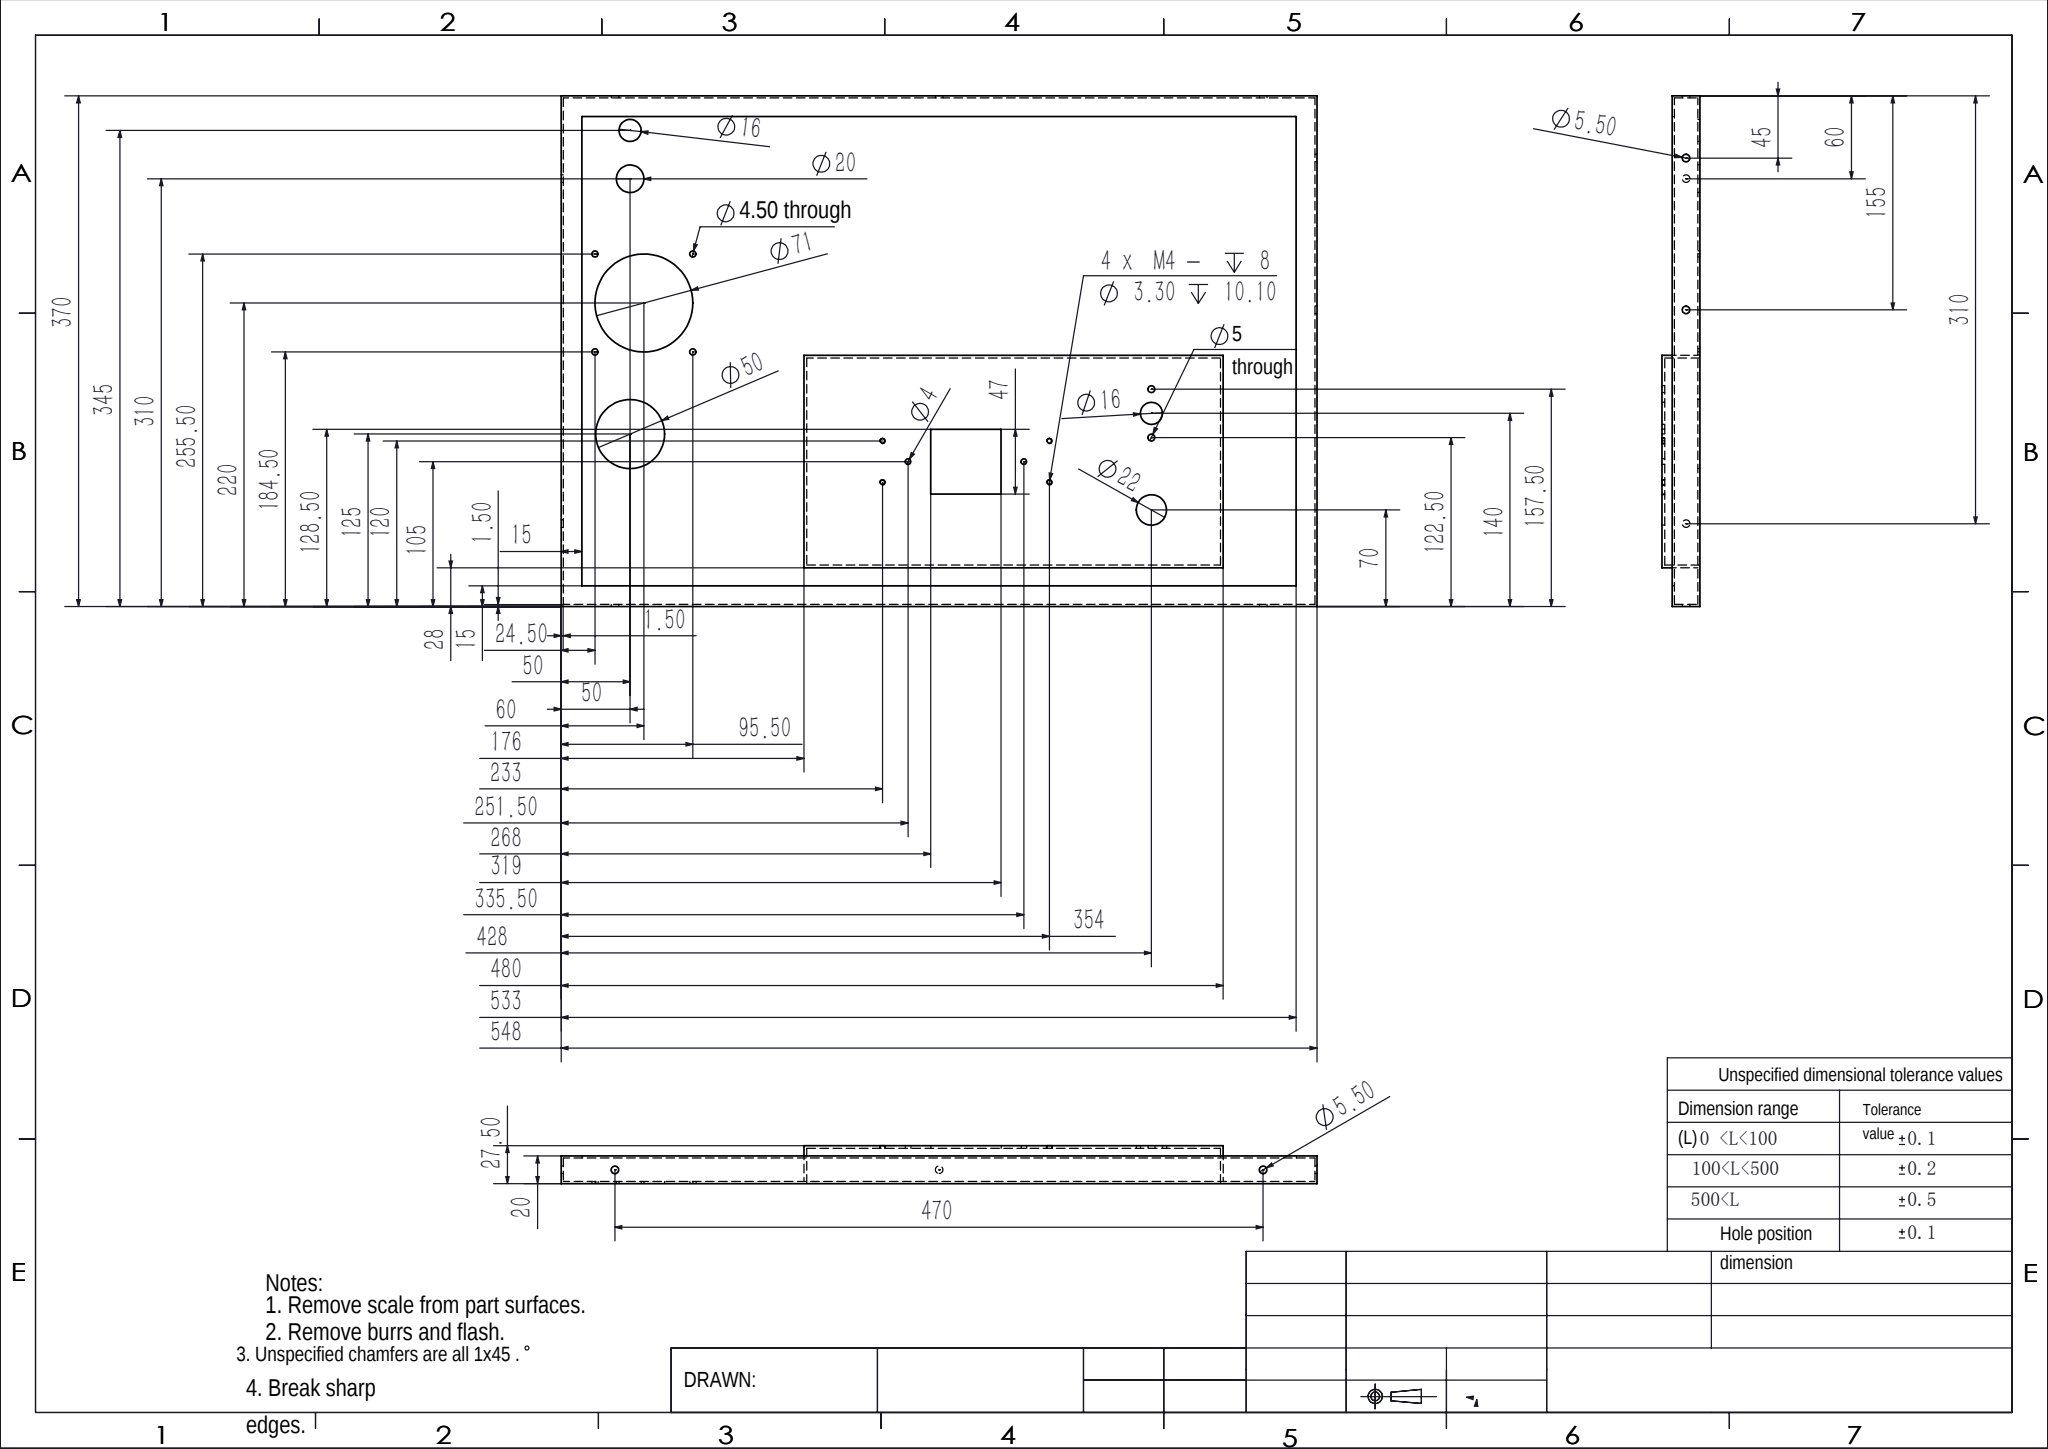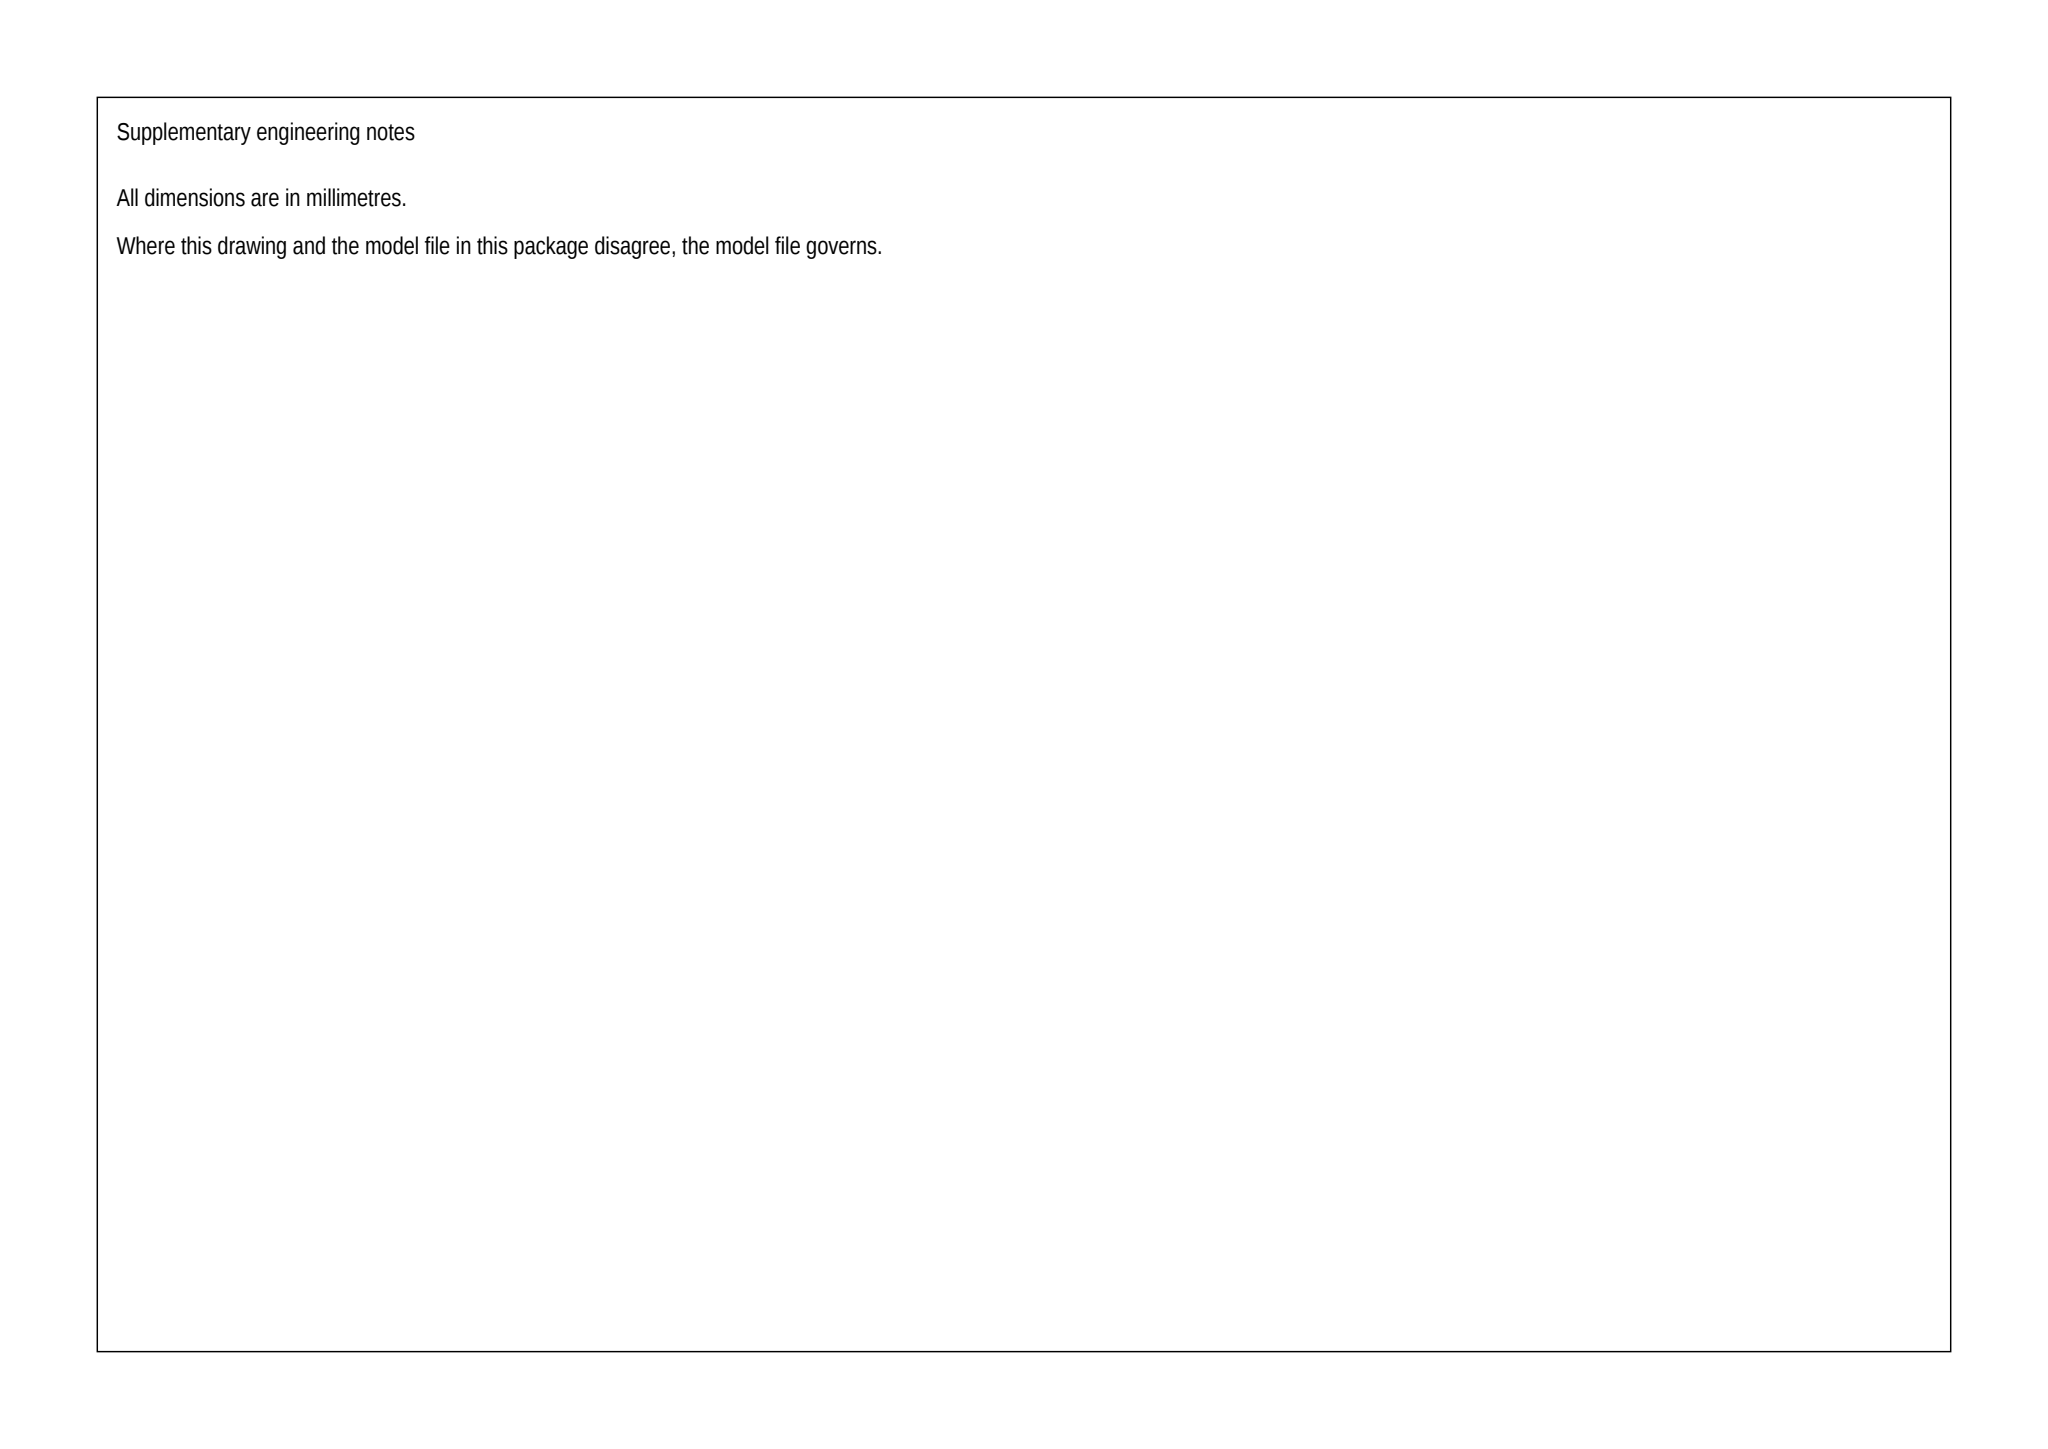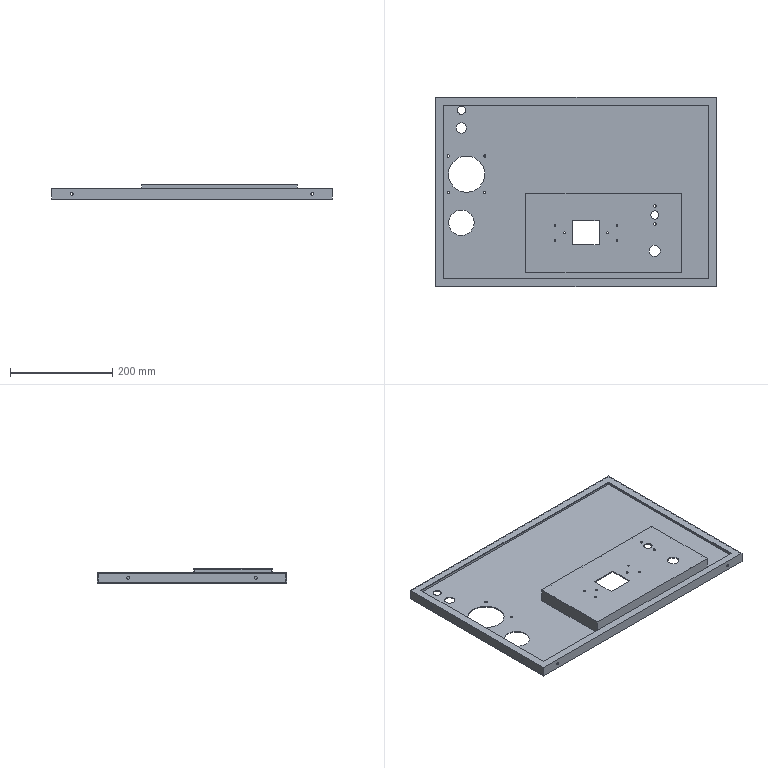Part | SolidWorks | mm | 1 solid | 84 faces | box 548 x 370 x 27.5 mm | volume 444254 mm3 | cylinder 54 | plane 30 | commonest cylinder face diameters 5.5 x18 3.3 x8 4.5 x8 4 x4 5 x4 16 x4 22 x2 71 x2
Drawing notes:
STEP 7.50 HIGH, 20 FACE TO 27.50 FACE, AT X178/480 & Y30/182 | from the solid: z planes 20 & 27.50 (diff 7.50); raised box bounded by x planes 178/480, y planes 30/182
RECESS OPEN AT BTM: 18.50 DP IN 20 THK AREA, 25.50 DP IN 27.50 AREA; ROOF 1.50/2 | from the solid: z planes 0/18.50/20 and 0/25.50/27.50: cavity open at bottom face z=0, roof 1.50 thk in main area, 2.0 thk under raised area
SQ CUTOUT 51 (X268-319) x 47 (Y81.50-128.50) THRU 2 THK TOP | from the solid: x planes 268 & 319 (51 wide), y planes 81.50 & 128.50 (47 high); top plate z25.50-27.50 = 2 thk; flanked by Ø4 holes at (251.50,105) & (335.50,105)
Ø5.50 THRU SIDE WALLS 1.50 THK AT X39, 274, 509; CL 10 FROM BTM | from the solid: cylinders Ø5.5 axis y at x=39, 274, 509, all z=10, length 1.5 (walls y0-1.5 & y368.5-370); 509-39=470 matches existing dim
build123d program:
from build123d import *

# Parameters (mm, degrees)
SKETCH1_W             = 548
SKETCH1_H             = 370
BOSS_EXTRUDE1_DEPTH   = 10
SKETCH6_W             = 518
SKETCH6_H             = 340
CUT_EXTRUDE2_DEPTH    = 5
SHELL1_T              = -1.5
SKETCH8_R             = 25
SKETCH8_R_2           = 10
SKETCH8_R_3           = 8
CUT_EXTRUDE4_DEPTH    = 10
SKETCH9_R             = 35.5
CUT_EXTRUDE5_DEPTH    = 10
SKETCH10_R            = 2.25
CUT_EXTRUDE6_DEPTH    = 10
SKETCH12_W            = 300
SKETCH12_H            = 150
CUT_EXTRUDE7_DEPTH    = 332.211
SKETCH13_W            = 304
SKETCH13_H            = 154
SKETCH13_W_2          = 300
SKETCH13_H_2          = 150
BOSS_EXTRUDE3_DEPTH   = 24
SKETCH14_W            = 304
SKETCH14_H            = 154
BOSS_EXTRUDE4_DEPTH   = 2
SKETCH15_R            = 11
SKETCH15_R_2          = 8
SKETCH15_W            = 51
SKETCH15_H            = 47
CUT_EXTRUDE8_DEPTH    = 332.589
SKETCH16_R            = 2.5
CUT_EXTRUDE9_DEPTH    = 332.589
SKETCH17_R            = 2
CUT_EXTRUDE10_DEPTH   = 332.589
SKETCH18_R            = 2.75
CUT_EXTRUDE11_DEPTH   = 2
CUT_EXTRUDE12_START   = -2
SKETCH19_R            = 2.75
CUT_EXTRUDE12_DEPTH   = 2
SKETCH20_R            = 2.75
CUT_EXTRUDE13_DEPTH   = 2
SKETCH21_R            = 2.75
CUT_EXTRUDE14_DEPTH   = 2
M4_TAPPED_HOLE1_D     = 3.3
M4_TAPPED_HOLE1_DEPTH = 10.1
M4_TAPPED_HOLE1_TIP   = 0.9914


with BuildPart() as part:
    # Sketch1 → Boss-Extrude1 (new, symmetric)
    with BuildSketch(Plane.XY):
        Rectangle(SKETCH1_W, SKETCH1_H)
    extrude(amount=BOSS_EXTRUDE1_DEPTH, both=True)

    # Sketch6 → Cut-Extrude2 (cut)
    with BuildSketch(Plane.XY.offset(10)):
        Rectangle(SKETCH6_W, SKETCH6_H)
    extrude(amount=-CUT_EXTRUDE2_DEPTH, mode=Mode.SUBTRACT)

    # Shell1
    shell1_openings = [part.faces().sort_by_distance(p)[0] for p in [
        (0, -170, 7.5),
        (-259, 0, 7.5),
        (0, 170, 7.5),
        (259, 0, 7.5),
        (0, 0, 5),
    ]]
    offset(amount=SHELL1_T, openings=shell1_openings, kind=Kind.INTERSECTION)

    # Sketch8 → Cut-Extrude4 (cut)
    with BuildSketch(Plane(origin=(0, 0, -10), x_dir=(-1, 0, 0), z_dir=(0, 0, -1))):
        with Locations((224, -60)):
            Circle(SKETCH8_R)
        with Locations((224, 125)):
            Circle(SKETCH8_R_2)
        with Locations((224, 160)):
            Circle(SKETCH8_R_3)
    extrude(amount=-CUT_EXTRUDE4_DEPTH, mode=Mode.SUBTRACT)

    # Sketch9 → Cut-Extrude5 (cut)
    with BuildSketch(Plane(origin=(0, 0, -10), x_dir=(-1, 0, 0), z_dir=(0, 0, -1))):
        with Locations((214, 35)):
            Circle(SKETCH9_R)
    extrude(amount=-CUT_EXTRUDE5_DEPTH, mode=Mode.SUBTRACT)

    # Sketch10 → Cut-Extrude6 (cut)
    with BuildSketch(Plane(origin=(0, 0, -10), x_dir=(-1, 0, 0), z_dir=(0, 0, -1))):
        with Locations((178.5, -0.5)):
            Circle(SKETCH10_R)
        with Locations((178.5, 70.5)):
            Circle(SKETCH10_R)
        with Locations((249.5, 70.5)):
            Circle(SKETCH10_R)
        with Locations((249.5, -0.5)):
            Circle(SKETCH10_R)
    extrude(amount=-CUT_EXTRUDE6_DEPTH, mode=Mode.SUBTRACT)

    # Sketch12 → Cut-Extrude7 (cut, through all)
    with BuildSketch(Plane(origin=(0, 0, -10), x_dir=(-1, 0, 0), z_dir=(0, 0, -1))):
        with Locations((-54, -80)):
            Rectangle(SKETCH12_W, SKETCH12_H)
    extrude(amount=-CUT_EXTRUDE7_DEPTH, mode=Mode.SUBTRACT)

    # Sketch13 → Boss-Extrude3 (add)
    with BuildSketch(Plane.XY.offset(-8.5)):
        with Locations((54, -80)):
            Rectangle(SKETCH13_W, SKETCH13_H)
        with Locations((54, -80)):
            Rectangle(SKETCH13_W_2, SKETCH13_H_2, mode=Mode.SUBTRACT)
    extrude(amount=BOSS_EXTRUDE3_DEPTH)

    # Sketch14 → Boss-Extrude4 (add)
    with BuildSketch(Plane.XY.offset(15.5)):
        with Locations((54, -80)):
            Rectangle(SKETCH14_W, SKETCH14_H)
    extrude(amount=BOSS_EXTRUDE4_DEPTH)

    # Sketch15 → Cut-Extrude8 (cut, through all)
    with BuildSketch(Plane(origin=(0, 0, 15.5), x_dir=(-1, 0, 0), z_dir=(0, 0, -1))):
        with Locations((-154, -115)):
            Circle(SKETCH15_R)
        with Locations((-154, -45)):
            Circle(SKETCH15_R_2)
        with Locations((-19.5, -80)):
            Rectangle(SKETCH15_W, SKETCH15_H)
    extrude(amount=-CUT_EXTRUDE8_DEPTH, mode=Mode.SUBTRACT)

    # Sketch16 → Cut-Extrude9 (cut, through all)
    with BuildSketch(Plane(origin=(0, 0, 15.5), x_dir=(-1, 0, 0), z_dir=(0, 0, -1))):
        with Locations((-154, -62.5)):
            Circle(SKETCH16_R)
        with Locations((-154, -27.5)):
            Circle(SKETCH16_R)
    extrude(amount=-CUT_EXTRUDE9_DEPTH, mode=Mode.SUBTRACT)

    # Sketch17 → Cut-Extrude10 (cut, through all)
    with BuildSketch(Plane(origin=(0, 0, 15.5), x_dir=(-1, 0, 0), z_dir=(0, 0, -1))):
        with Locations((22.5, -80)):
            Circle(SKETCH17_R)
        with Locations((-61.5, -80)):
            Circle(SKETCH17_R)
    extrude(amount=-CUT_EXTRUDE10_DEPTH, mode=Mode.SUBTRACT)

    # Sketch18 → Cut-Extrude11 (cut)
    with BuildSketch(Plane(origin=(0, 185, 0), x_dir=(1, 0, 0), z_dir=(0, 1, 0))):
        with Locations(Location((0, 0, 0), (0, 0, 270))):
            Circle(SKETCH18_R)
        with Locations(Location((-235, 0, 0), (0, 0, 270))):
            Circle(SKETCH18_R)
        with Locations(Location((235, 0, 0), (0, 0, 90))):
            Circle(SKETCH18_R)
    extrude(amount=-CUT_EXTRUDE11_DEPTH, mode=Mode.SUBTRACT)

    # Sketch19 → Cut-Extrude12 (cut)
    with BuildSketch(Plane.XZ.offset(185).offset(CUT_EXTRUDE12_START)):
        with Locations(Location((235, 0, 0), (0, 0, 270))):
            Circle(SKETCH19_R)
        with Locations(Location((-235, 0, 0), (0, 0, 90))):
            Circle(SKETCH19_R)
    extrude(amount=CUT_EXTRUDE12_DEPTH, mode=Mode.SUBTRACT)

    # Sketch20 → Cut-Extrude13 (cut)
    with BuildSketch(Plane.ZY.offset(274)):
        with Locations((0, 125)):
            Circle(SKETCH20_R)
        with Locations(Location((0, -125, 0), (0, 0, 180))):
            Circle(SKETCH20_R)
    extrude(amount=-CUT_EXTRUDE13_DEPTH, mode=Mode.SUBTRACT)

    # Sketch21 → Cut-Extrude14 (cut)
    with BuildSketch(Plane(origin=(274, 0, 0), x_dir=(0, 0, -1), z_dir=(1, 0, 0))):
        with Locations(Location((0, 140, 0), (0, 0, 90))):
            Circle(SKETCH21_R)
        with Locations(Location((0, 30, 0), (0, 0, 90))):
            Circle(SKETCH21_R)
    extrude(amount=-CUT_EXTRUDE14_DEPTH, mode=Mode.SUBTRACT)

    # M4 Tapped Hole1
    with Locations(Plane(origin=(0, 0, 15.5), x_dir=(-1, 0, 0), z_dir=(0, 0, -1))):
        with Locations((41, -95), (41, -65), (-80, -65), (-80, -95)):
            Hole(M4_TAPPED_HOLE1_D / 2, depth=M4_TAPPED_HOLE1_DEPTH)
            with Locations((0, 0, -(M4_TAPPED_HOLE1_DEPTH + M4_TAPPED_HOLE1_TIP / 2))):  # 118° drill point
                Cone(0, M4_TAPPED_HOLE1_D / 2, M4_TAPPED_HOLE1_TIP, mode=Mode.SUBTRACT)


solid = part.part